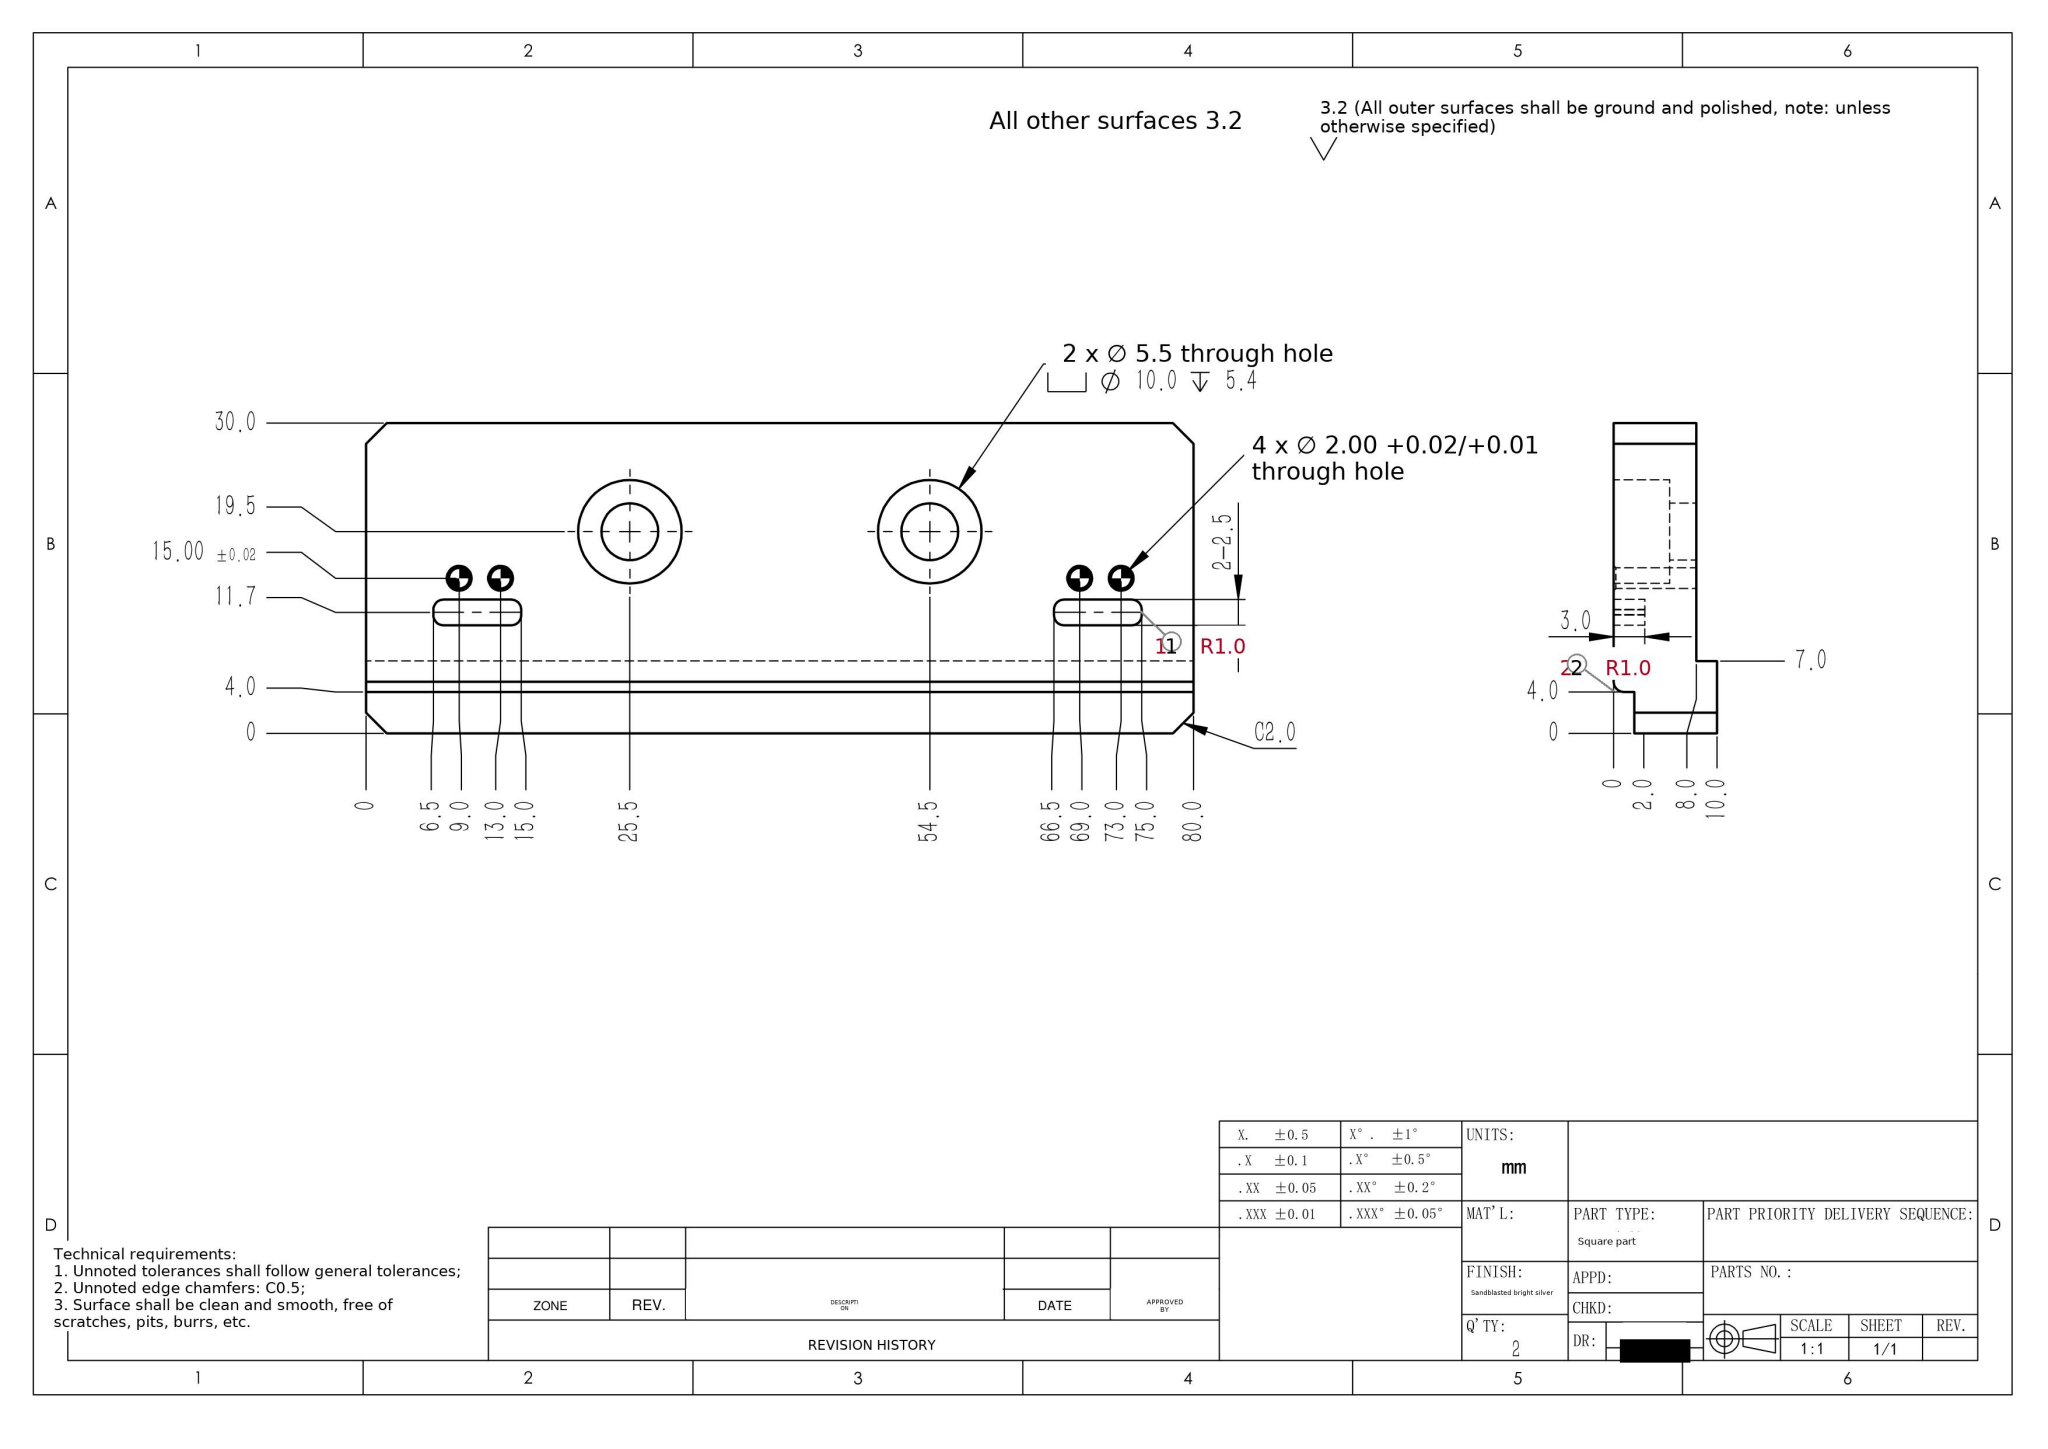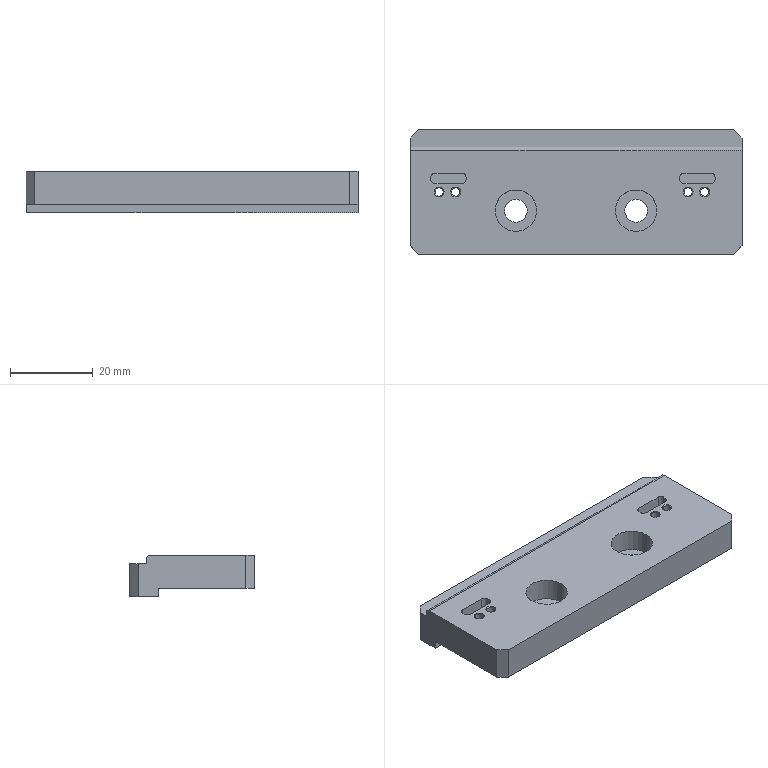Part | SolidWorks | mm | 1 solid | 59 faces | box 80 x 30 x 10 mm | volume 18404 mm3 | plane 26 | cylinder 25 | cone 8 | commonest cylinder face diameters 2 x17 10 x4 5.5 x4
build123d program:
from build123d import *

# Parameters (mm, degrees)
SKETCH1_W                                       = 80
SKETCH1_H                                       = 30
BOSS_EXTRUDE1_DEPTH                             = 10
SKETCH2_W                                       = 80
SKETCH2_H                                       = 4
CUT_EXTRUDE1_DEPTH                              = 2
M5_HEX_SOCKET_HEAD_CAP_SCREW_CBORE1_D           = 5.5
M5_HEX_SOCKET_HEAD_CAP_SCREW_CBORE1_CBORE_D     = 10
M5_HEX_SOCKET_HEAD_CAP_SCREW_CBORE1_CBORE_DEPTH = 5.4
SIZE_MM_DOWEL_PIN_HOLE1_D                       = 2
SKETCH7_W                                       = 8.5
SKETCH7_H                                       = 2.5
CUT_EXTRUDE2_DEPTH                              = 3
FILLET1_R                                       = 1
LPATTERN1_COUNT                                 = 2
LPATTERN1_PITCH                                 = 60
FILLET1_OF_LPATTERN1_R                          = 1
SKETCH8_W                                       = 80
SKETCH8_H                                       = 23
CUT_EXTRUDE3_DEPTH                              = 2
CHAMFER1_SIZE                                   = 2
CHAMFER2_SIZE                                   = 0.2
FILLET2_R                                       = 1


with BuildPart() as part:
    # Sketch1 → Boss-Extrude1 (new body)
    with BuildSketch(Plane.XY):
        with Locations((0, 15)):
            Rectangle(SKETCH1_W, SKETCH1_H)
    extrude(amount=BOSS_EXTRUDE1_DEPTH)

    # Sketch2 → Cut-Extrude1 (cut)
    with BuildSketch(Plane.XY.offset(10)):
        with Locations((0, 28)):
            Rectangle(SKETCH2_W, SKETCH2_H)
    extrude(amount=-CUT_EXTRUDE1_DEPTH, mode=Mode.SUBTRACT)

    # M5 Hex Socket Head Cap Screw CBORE1 (through all)
    with Locations(Plane.XY.offset(10)):
        with Locations((-14.5, 10.5), (14.5, 10.5)):
            CounterBoreHole(M5_HEX_SOCKET_HEAD_CAP_SCREW_CBORE1_D / 2, M5_HEX_SOCKET_HEAD_CAP_SCREW_CBORE1_CBORE_D / 2, M5_HEX_SOCKET_HEAD_CAP_SCREW_CBORE1_CBORE_DEPTH)

    # Size mm Dowel Pin Hole1 (through all)
    with Locations(Plane.XY.offset(10)):
        with Locations((-33, 15), (-29, 15)):
            size_mm_dowel_pin_hole1 = Hole(SIZE_MM_DOWEL_PIN_HOLE1_D / 2)

    # Sketch7 → Cut-Extrude2 (cut)
    with BuildSketch(Plane.XY.offset(10)):
        with Locations((-30.75, 18.3)):
            Rectangle(SKETCH7_W, SKETCH7_H)
    cut_extrude2 = extrude(amount=-CUT_EXTRUDE2_DEPTH, mode=Mode.SUBTRACT)

    # Fillet1
    fillet1_edges = [part.edges().sort_by_distance(p)[0] for p in [
        (-35, 17.05, 8.5),
        (-35, 19.55, 8.5),
        (-26.5, 19.55, 8.5),
        (-26.5, 17.05, 8.5),
    ]]
    fillet(fillet1_edges, radius=FILLET1_R)

    # LPattern1: Size mm Dowel Pin Hole1, Cut-Extrude2 ×2
    with Locations(*[(i * LPATTERN1_PITCH, 0, 0) for i in range(1, LPATTERN1_COUNT)]):
        add(size_mm_dowel_pin_hole1, mode=Mode.SUBTRACT)
        add(cut_extrude2, mode=Mode.SUBTRACT)

    # Fillet1 of LPattern1
    fillet1_of_lpattern1_edges = [part.edges().sort_by_distance(p)[0] for p in [
        (25, 17.05, 8.5),
        (25, 19.55, 8.5),
        (33.5, 19.55, 8.5),
        (33.5, 17.05, 8.5),
    ]]
    fillet(fillet1_of_lpattern1_edges, radius=FILLET1_OF_LPATTERN1_R)

    # Sketch8 → Cut-Extrude3 (cut)
    with BuildSketch(Plane(origin=(0, 0, 0), x_dir=(-1, 0, 0), z_dir=(0, 0, -1))):
        with Locations((0, 11.5)):
            Rectangle(SKETCH8_W, SKETCH8_H)
    extrude(amount=-CUT_EXTRUDE3_DEPTH, mode=Mode.SUBTRACT)

    # Chamfer1
    chamfer1_edges = [part.edges().sort_by_distance(p)[0] for p in [
        (-40, 30, 4),
        (40, 30, 4),
        (40, 0, 6),
        (-40, 0, 6),
    ]]
    chamfer(chamfer1_edges, length=CHAMFER1_SIZE)

    # Chamfer2
    chamfer2_edges = [part.edges().sort_by_distance(p)[0] for p in [
        (-28, 15, 10),
        (-32, 15, 10),
        (28, 15, 10),
        (32, 15, 10),
    ]]
    chamfer(chamfer2_edges, length=CHAMFER2_SIZE)

    # Fillet2
    fillet2_edges = [part.edges().sort_by_distance(p)[0] for p in [
        (0, 26, 10),
    ]]
    fillet(fillet2_edges, radius=FILLET2_R)


solid = part.part